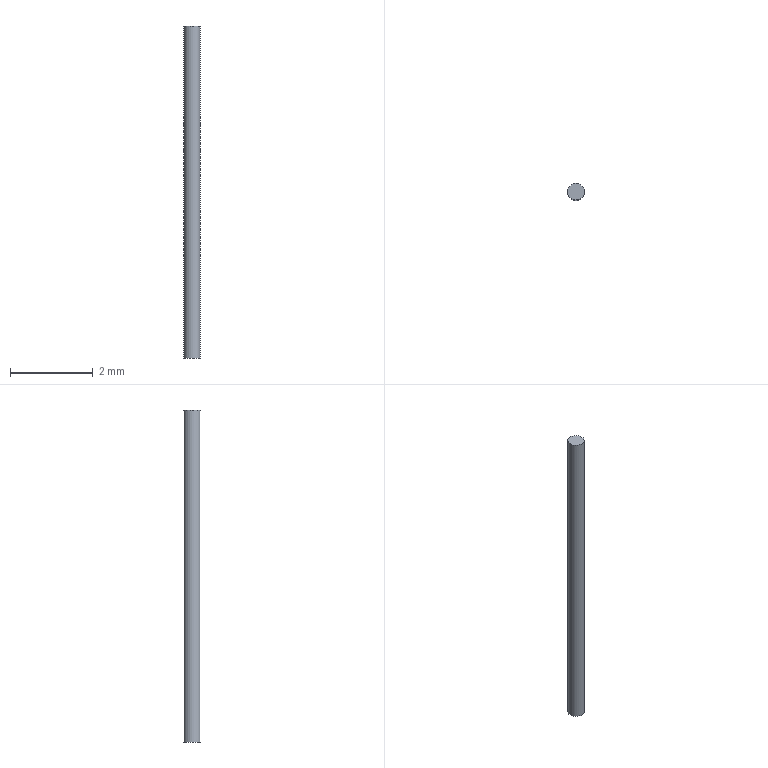Component | NX | PIN | 1 solid | 3 faces | box 0.4 x 0.4 x 8 mm | volume 1 mm3 | plane 2 | cylinder 1 | commonest cylinder face diameters 0.4 x1
STEP:
#1=CARTESIAN_POINT('',(0.,0.,0.));
#2=DIRECTION('',(0.,0.,1.));
#3=DIRECTION('',(1.,0.,0.));
#4=AXIS2_PLACEMENT_3D('',#1,#2,#3);
#5=CARTESIAN_POINT('',(-0.5644,-1.425,-10.756));
#6=VERTEX_POINT('',#5);
#7=CARTESIAN_POINT('',(-0.7644,-1.425,-10.756));
#8=DIRECTION('',(0.,0.,1.));
#9=DIRECTION('',(1.,0.,0.));
#10=AXIS2_PLACEMENT_3D('',#7,#8,#9);
#11=CIRCLE('',#10,0.2);
#12=CARTESIAN_POINT('',(-0.7644,-1.425,-10.756));
#13=DIRECTION('',(0.,0.,-1.));
#14=DIRECTION('',(-1.,0.,0.));
#15=AXIS2_PLACEMENT_3D('',#12,#13,#14);
#16=CYLINDRICAL_SURFACE('',#15,0.2);
#17=CARTESIAN_POINT('',(9.425,0.));
#18=DIRECTION('',(-1.,0.));
#19=VECTOR('',#18,1.);
#20=LINE('',#17,#19);
#21=(GEOMETRIC_REPRESENTATION_CONTEXT(2)PARAMETRIC_REPRESENTATION_CONTEXT()REPRESENTATION_CONTEXT('',''));
#22=DEFINITIONAL_REPRESENTATION('',(#20),#21);
#23=PCURVE('',#16,#22);
#24=CARTESIAN_POINT('',(-0.7644,-1.425,-10.756));
#25=DIRECTION('',(0.,0.,1.));
#26=DIRECTION('',(1.,0.,0.));
#27=AXIS2_PLACEMENT_3D('',#24,#25,#26);
#28=PLANE('',#27);
#29=CARTESIAN_POINT('',(0.,0.));
#30=DIRECTION('',(1.,0.));
#31=AXIS2_PLACEMENT_2D('',#29,#30);
#32=CIRCLE('',#31,0.2);
#33=(GEOMETRIC_REPRESENTATION_CONTEXT(2)PARAMETRIC_REPRESENTATION_CONTEXT()REPRESENTATION_CONTEXT('',''));
#34=DEFINITIONAL_REPRESENTATION('',(#32),#33);
#35=PCURVE('',#28,#34);
#36=SURFACE_CURVE('',#11,(#23,#35),.PCURVE_S1.);
#37=EDGE_CURVE('',#6,#6,#36,.T.);
#38=ORIENTED_EDGE('',*,*,#37,.F.);
#39=CARTESIAN_POINT('',(-0.5644,-1.425,-18.756));
#40=VERTEX_POINT('',#39);
#41=CARTESIAN_POINT('',(-0.5644,-1.425,-10.756));
#42=CARTESIAN_POINT('',(-0.5644,-1.425,-18.756));
#43=B_SPLINE_CURVE_WITH_KNOTS('',1,(#41,#42),.UNSPECIFIED.,.F.,.F.,(2,2),(0.,8.),.PIECEWISE_BEZIER_KNOTS.);
#44=CARTESIAN_POINT('',(9.425,0.));
#45=DIRECTION('',(0.,1.));
#46=VECTOR('',#45,1.);
#47=LINE('',#44,#46);
#48=(GEOMETRIC_REPRESENTATION_CONTEXT(2)PARAMETRIC_REPRESENTATION_CONTEXT()REPRESENTATION_CONTEXT('',''));
#49=DEFINITIONAL_REPRESENTATION('',(#47),#48);
#50=PCURVE('',#16,#49);
#51=CARTESIAN_POINT('',(3.142,0.));
#52=DIRECTION('',(0.,1.));
#53=VECTOR('',#52,1.);
#54=LINE('',#51,#53);
#55=(GEOMETRIC_REPRESENTATION_CONTEXT(2)PARAMETRIC_REPRESENTATION_CONTEXT()REPRESENTATION_CONTEXT('',''));
#56=DEFINITIONAL_REPRESENTATION('',(#54),#55);
#57=PCURVE('',#16,#56);
#58=SEAM_CURVE('',#43,(#50,#57),.PCURVE_S1.);
#59=EDGE_CURVE('',#6,#40,#58,.T.);
#60=ORIENTED_EDGE('',*,*,#59,.T.);
#61=CARTESIAN_POINT('',(-0.7644,-1.425,-18.756));
#62=DIRECTION('',(0.,0.,1.));
#63=DIRECTION('',(1.,0.,0.));
#64=AXIS2_PLACEMENT_3D('',#61,#62,#63);
#65=CIRCLE('',#64,0.2);
#66=CARTESIAN_POINT('',(9.425,8.));
#67=DIRECTION('',(-1.,0.));
#68=VECTOR('',#67,1.);
#69=LINE('',#66,#68);
#70=(GEOMETRIC_REPRESENTATION_CONTEXT(2)PARAMETRIC_REPRESENTATION_CONTEXT()REPRESENTATION_CONTEXT('',''));
#71=DEFINITIONAL_REPRESENTATION('',(#69),#70);
#72=PCURVE('',#16,#71);
#73=CARTESIAN_POINT('',(-0.7644,-1.425,-18.756));
#74=DIRECTION('',(0.,0.,1.));
#75=DIRECTION('',(1.,0.,0.));
#76=AXIS2_PLACEMENT_3D('',#73,#74,#75);
#77=PLANE('',#76);
#78=CARTESIAN_POINT('',(0.,0.));
#79=DIRECTION('',(1.,0.));
#80=AXIS2_PLACEMENT_2D('',#78,#79);
#81=CIRCLE('',#80,0.2);
#82=(GEOMETRIC_REPRESENTATION_CONTEXT(2)PARAMETRIC_REPRESENTATION_CONTEXT()REPRESENTATION_CONTEXT('',''));
#83=DEFINITIONAL_REPRESENTATION('',(#81),#82);
#84=PCURVE('',#77,#83);
#85=SURFACE_CURVE('',#65,(#72,#84),.PCURVE_S1.);
#86=EDGE_CURVE('',#40,#40,#85,.T.);
#87=ORIENTED_EDGE('',*,*,#86,.T.);
#88=ORIENTED_EDGE('',*,*,#59,.F.);
#89=EDGE_LOOP('',(#38,#60,#87,#88));
#90=FACE_BOUND('',#89,.T.);
#91=ADVANCED_FACE('',(#90),#16,.T.);
#92=ORIENTED_EDGE('',*,*,#37,.T.);
#93=EDGE_LOOP('',(#92));
#94=FACE_BOUND('',#93,.T.);
#95=ADVANCED_FACE('',(#94),#28,.T.);
#96=ORIENTED_EDGE('',*,*,#86,.F.);
#97=EDGE_LOOP('',(#96));
#98=FACE_BOUND('',#97,.T.);
#99=ADVANCED_FACE('',(#98),#77,.F.);
#100=CLOSED_SHELL('',(#91,#95,#99));
#101=MANIFOLD_SOLID_BREP('',#100);
#102=(LENGTH_UNIT()NAMED_UNIT(*)SI_UNIT(.MILLI.,.METRE.));
#103=UNCERTAINTY_MEASURE_WITH_UNIT(LENGTH_MEASURE(0.00001),#102,'','');
#104=(NAMED_UNIT(*)PLANE_ANGLE_UNIT()SI_UNIT($,.RADIAN.));
#105=(NAMED_UNIT(*)SI_UNIT($,.STERADIAN.)SOLID_ANGLE_UNIT());
#106=(GEOMETRIC_REPRESENTATION_CONTEXT(3)GLOBAL_UNCERTAINTY_ASSIGNED_CONTEXT((#103))GLOBAL_UNIT_ASSIGNED_CONTEXT((#102,#104,#105))REPRESENTATION_CONTEXT('',''));
#107=ADVANCED_BREP_SHAPE_REPRESENTATION('',(#4,#101),#106);